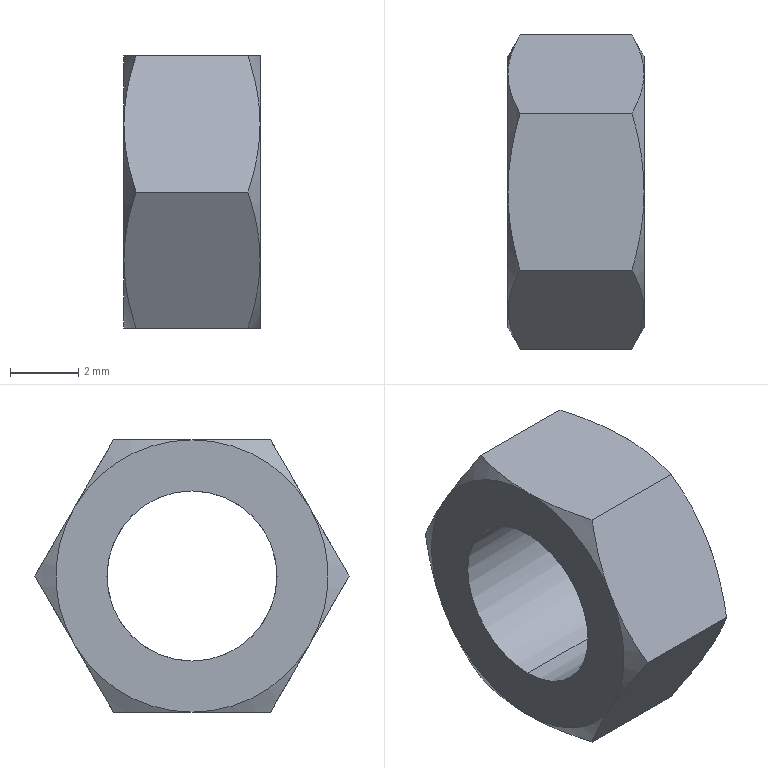Component | SolidWorks | 17268PB16x60SU(58)+(CS1-M-2)-1_17268164nut1-1 | 1 solid | 22 faces | box 4 x 9.24 x 8 mm | volume 142 mm3 | cone 12 | plane 8 | cylinder 2 | commonest cylinder face diameters 5 x2
build123d program:
from build123d import *

# Parameters (mm, degrees)
CUT_EXTRUDE1_DEPTH              = 2
CUT_EXTRUDE1_DEPTH_BACK         = 2
SKETCH3_W                       = 16
SKETCH3_H                       = 16
THREAD_FIT_RELIEF_M5_DEPTH      = 8.303
THREAD_FIT_RELIEF_M5_DEPTH_BACK = 8.303
SKETCH1_R                       = 2.5


with BuildPart() as part:
    # Sketch1_2 → Revolve1 (revolve)
    with BuildSketch(Plane.XY, mode=Mode.PRIVATE) as revolve1_sk:
        Polygon((-2, 0), (-2, 4), (-1.538, 4.8), (1.538, 4.8), (2, 4), (2, 0), align=None)
    revolve(revolve1_sk.sketch.rotate(Axis((2, 0, 0), (-1, 0, 0)), 270), axis=Axis((2, 0, 0), (-1, 0, 0)))

    # Sketch2 → Cut-Revolve1 (revolve, cut)
    with BuildSketch(Plane.XY, mode=Mode.PRIVATE) as cut_revolve1_sk:
        Polygon((-2, 0), (-2, 2.5), (-1.567, 2.067), (1.567, 2.067), (2, 2.5), (2, 0), align=None)
    revolve(cut_revolve1_sk.sketch.rotate(Axis((2, 0, 0), (-1, 0, 0)), 270), axis=Axis((2, 0, 0), (-1, 0, 0)), mode=Mode.SUBTRACT)

    # Sketch3 → Cut-Extrude1 (cut, two sides: drawn at the far end of the back side and taken through both)
    with BuildSketch(Plane(origin=(0, 0, 0), x_dir=(0, 0, -1), z_dir=(1, 0, 0)).offset(-CUT_EXTRUDE1_DEPTH_BACK)):
        Rectangle(SKETCH3_W, SKETCH3_H)
        Polygon((-4, -2.309), (0, -4.619), (4, -2.309), (4, 2.309), (0, 4.619), (-4, 2.309), align=None, mode=Mode.SUBTRACT)
    extrude(amount=CUT_EXTRUDE1_DEPTH + CUT_EXTRUDE1_DEPTH_BACK, mode=Mode.SUBTRACT)

    # Sketch1 → Thread fit relief M5 (cut, two sides: drawn at the far end of the back side and taken through both)
    with BuildSketch(Plane.ZY.offset(2).offset(-THREAD_FIT_RELIEF_M5_DEPTH_BACK)):
        Circle(SKETCH1_R)
    extrude(amount=THREAD_FIT_RELIEF_M5_DEPTH + THREAD_FIT_RELIEF_M5_DEPTH_BACK, mode=Mode.SUBTRACT)


solid = part.part

# Placed as in the assembly
solid = solid.moved(Location((-2.6, -27.579, 21.5), (0, 0, 0)))
STEP:
#1=CARTESIAN_POINT('',(-0.1811,-1.086,0.9449));
#2=VERTEX_POINT('',#1);
#3=CARTESIAN_POINT('',(-0.1811,-1.086,0.748));
#4=VERTEX_POINT('',#3);
#5=CARTESIAN_POINT('',(-0.1811,-1.086,0.8465));
#6=DIRECTION('',(1.,-0.,-0.));
#7=DIRECTION('',(0.,0.,-1.));
#8=AXIS2_PLACEMENT_3D('',#5,#6,#7);
#9=CIRCLE('',#8,0.09843);
#10=EDGE_CURVE('',#2,#4,#9,.T.);
#11=ORIENTED_EDGE('',*,*,#10,.F.);
#12=CARTESIAN_POINT('',(-0.02362,-1.086,0.9449));
#13=VERTEX_POINT('',#12);
#14=CARTESIAN_POINT('',(-0.1811,-1.086,0.9449));
#15=DIRECTION('',(1.,-0.,-0.));
#16=VECTOR('',#15,39.37);
#17=LINE('',#14,#16);
#18=EDGE_CURVE('',#2,#13,#17,.T.);
#19=ORIENTED_EDGE('',*,*,#18,.T.);
#20=CARTESIAN_POINT('',(-0.02362,-1.086,0.748));
#21=VERTEX_POINT('',#20);
#22=CARTESIAN_POINT('',(-0.02362,-1.086,0.9449));
#23=CARTESIAN_POINT('',(-0.02362,-1.099,0.9449));
#24=CARTESIAN_POINT('',(-0.02362,-1.112,0.9423));
#25=CARTESIAN_POINT('',(-0.02362,-1.135,0.9325));
#26=CARTESIAN_POINT('',(-0.02362,-1.146,0.9252));
#27=CARTESIAN_POINT('',(-0.02362,-1.165,0.9069));
#28=CARTESIAN_POINT('',(-0.02362,-1.172,0.896));
#29=CARTESIAN_POINT('',(-0.02362,-1.182,0.8722));
#30=CARTESIAN_POINT('',(-0.02362,-1.184,0.8593));
#31=CARTESIAN_POINT('',(-0.02362,-1.184,0.8336));
#32=CARTESIAN_POINT('',(-0.02362,-1.182,0.8207));
#33=CARTESIAN_POINT('',(-0.02362,-1.172,0.7969));
#34=CARTESIAN_POINT('',(-0.02362,-1.165,0.786));
#35=CARTESIAN_POINT('',(-0.02362,-1.146,0.7677));
#36=CARTESIAN_POINT('',(-0.02362,-1.135,0.7605));
#37=CARTESIAN_POINT('',(-0.02362,-1.112,0.7506));
#38=CARTESIAN_POINT('',(-0.02362,-1.099,0.748));
#39=CARTESIAN_POINT('',(-0.02362,-1.086,0.748));
#40=B_SPLINE_CURVE_WITH_KNOTS('',3,(#22,#23,#24,#25,#26,#27,#28,#29,#30,#31,#32,#33,#34,#35,#36,#37,#38,#39),.UNSPECIFIED.,.F.,.F.,(4,2,2,2,2,2,2,2,4),(0.5,0.5625,0.625,0.6875,0.75,0.8125,0.875,0.9375,1.),.UNSPECIFIED.);
#41=EDGE_CURVE('',#13,#21,#40,.T.);
#42=ORIENTED_EDGE('',*,*,#41,.T.);
#43=CARTESIAN_POINT('',(-0.1811,-1.086,0.748));
#44=DIRECTION('',(1.,-0.,-0.));
#45=VECTOR('',#44,39.37);
#46=LINE('',#43,#45);
#47=EDGE_CURVE('',#4,#21,#46,.T.);
#48=ORIENTED_EDGE('',*,*,#47,.F.);
#49=EDGE_LOOP('',(#11,#19,#42,#48));
#50=FACE_OUTER_BOUND('',#49,.T.);
#51=CARTESIAN_POINT('',(-0.1811,-1.086,0.8465));
#52=DIRECTION('',(1.,-0.,-0.));
#53=DIRECTION('',(0.,0.,-1.));
#54=AXIS2_PLACEMENT_3D('',#51,#52,#53);
#55=CYLINDRICAL_SURFACE('',#54,0.09843);
#56=ADVANCED_FACE('',(#50),#55,.F.);
#57=CARTESIAN_POINT('',(-0.03769,-0.9949,1.004));
#58=VERTEX_POINT('',#57);
#59=CARTESIAN_POINT('',(-0.02362,-0.9494,0.9252));
#60=VERTEX_POINT('',#59);
#61=CARTESIAN_POINT('',(-0.03769,-0.9949,1.004));
#62=CARTESIAN_POINT('',(-0.0291,-0.98,0.9782));
#63=CARTESIAN_POINT('',(-0.02362,-0.9649,0.952));
#64=CARTESIAN_POINT('',(-0.02362,-0.9494,0.9252));
#65=B_SPLINE_CURVE_WITH_KNOTS('',3,(#61,#62,#63,#64),.UNSPECIFIED.,.F.,.F.,(4,4),(0.00000024,0.002337),.UNSPECIFIED.);
#66=EDGE_CURVE('',#58,#60,#65,.T.);
#67=ORIENTED_EDGE('',*,*,#66,.F.);
#68=CARTESIAN_POINT('',(-0.02362,-1.086,1.004));
#69=VERTEX_POINT('',#68);
#70=CARTESIAN_POINT('',(-0.02362,-1.086,1.004));
#71=CARTESIAN_POINT('',(-0.02362,-1.07,1.004));
#72=CARTESIAN_POINT('',(-0.02498,-1.055,1.004));
#73=CARTESIAN_POINT('',(-0.02991,-1.024,1.004));
#74=CARTESIAN_POINT('',(-0.03344,-1.01,1.004));
#75=CARTESIAN_POINT('',(-0.03769,-0.9949,1.004));
#76=B_SPLINE_CURVE_WITH_KNOTS('',3,(#70,#71,#72,#73,#74,#75),.UNSPECIFIED.,.F.,.F.,(4,2,4),(0.006473,0.007642,0.008811),.UNSPECIFIED.);
#77=EDGE_CURVE('',#69,#58,#76,.T.);
#78=ORIENTED_EDGE('',*,*,#77,.F.);
#79=CARTESIAN_POINT('',(-0.02362,-1.086,0.8465));
#80=DIRECTION('',(1.,-0.,-0.));
#81=DIRECTION('',(-0.,0.,-1.));
#82=AXIS2_PLACEMENT_3D('',#79,#80,#81);
#83=CIRCLE('',#82,0.1575);
#84=EDGE_CURVE('',#60,#69,#83,.T.);
#85=ORIENTED_EDGE('',*,*,#84,.F.);
#86=EDGE_LOOP('',(#67,#78,#85));
#87=FACE_OUTER_BOUND('',#86,.T.);
#88=CARTESIAN_POINT('',(-0.04181,-1.086,0.8465));
#89=DIRECTION('',(-1.,0.,0.));
#90=DIRECTION('',(0.,0.,1.));
#91=AXIS2_PLACEMENT_3D('',#88,#89,#90);
#92=CONICAL_SURFACE('',#91,0.189,1.047);
#93=ADVANCED_FACE('',(#87),#92,.T.);
#94=CARTESIAN_POINT('',(-0.03769,-0.904,0.8465));
#95=VERTEX_POINT('',#94);
#96=CARTESIAN_POINT('',(-0.02362,-0.9494,0.9252));
#97=CARTESIAN_POINT('',(-0.02362,-0.9417,0.9118));
#98=CARTESIAN_POINT('',(-0.02497,-0.934,0.8985));
#99=CARTESIAN_POINT('',(-0.02987,-0.9189,0.8723));
#100=CARTESIAN_POINT('',(-0.0334,-0.9114,0.8593));
#101=CARTESIAN_POINT('',(-0.03769,-0.904,0.8465));
#102=B_SPLINE_CURVE_WITH_KNOTS('',3,(#96,#97,#98,#99,#100,#101),.UNSPECIFIED.,.F.,.F.,(4,2,4),(0.002337,0.003501,0.004665),.UNSPECIFIED.);
#103=EDGE_CURVE('',#60,#95,#102,.T.);
#104=ORIENTED_EDGE('',*,*,#103,.F.);
#105=CARTESIAN_POINT('',(-0.02362,-0.9494,0.7677));
#106=VERTEX_POINT('',#105);
#107=CARTESIAN_POINT('',(-0.02362,-1.086,0.8465));
#108=DIRECTION('',(1.,-0.,-0.));
#109=DIRECTION('',(-0.,0.,-1.));
#110=AXIS2_PLACEMENT_3D('',#107,#108,#109);
#111=CIRCLE('',#110,0.1575);
#112=EDGE_CURVE('',#106,#60,#111,.T.);
#113=ORIENTED_EDGE('',*,*,#112,.F.);
#114=CARTESIAN_POINT('',(-0.03769,-0.904,0.8465));
#115=CARTESIAN_POINT('',(-0.0291,-0.9188,0.8207));
#116=CARTESIAN_POINT('',(-0.02362,-0.9339,0.7945));
#117=CARTESIAN_POINT('',(-0.02362,-0.9494,0.7677));
#118=B_SPLINE_CURVE_WITH_KNOTS('',3,(#114,#115,#116,#117),.UNSPECIFIED.,.F.,.F.,(4,4),(0.00000024,0.002337),.UNSPECIFIED.);
#119=EDGE_CURVE('',#95,#106,#118,.T.);
#120=ORIENTED_EDGE('',*,*,#119,.F.);
#121=EDGE_LOOP('',(#104,#113,#120));
#122=FACE_OUTER_BOUND('',#121,.T.);
#123=CARTESIAN_POINT('',(-0.04181,-1.086,0.8465));
#124=DIRECTION('',(-1.,0.,0.));
#125=DIRECTION('',(0.,0.,1.));
#126=AXIS2_PLACEMENT_3D('',#123,#124,#125);
#127=CONICAL_SURFACE('',#126,0.189,1.047);
#128=ADVANCED_FACE('',(#122),#127,.T.);
#129=CARTESIAN_POINT('',(-0.03769,-0.9949,0.689));
#130=VERTEX_POINT('',#129);
#131=CARTESIAN_POINT('',(-0.02362,-0.9494,0.7677));
#132=CARTESIAN_POINT('',(-0.02362,-0.9571,0.7544));
#133=CARTESIAN_POINT('',(-0.02497,-0.9648,0.741));
#134=CARTESIAN_POINT('',(-0.02987,-0.98,0.7148));
#135=CARTESIAN_POINT('',(-0.0334,-0.9875,0.7018));
#136=CARTESIAN_POINT('',(-0.03769,-0.9949,0.689));
#137=B_SPLINE_CURVE_WITH_KNOTS('',3,(#131,#132,#133,#134,#135,#136),.UNSPECIFIED.,.F.,.F.,(4,2,4),(0.002337,0.003501,0.004665),.UNSPECIFIED.);
#138=EDGE_CURVE('',#106,#130,#137,.T.);
#139=ORIENTED_EDGE('',*,*,#138,.F.);
#140=CARTESIAN_POINT('',(-0.02362,-1.086,0.689));
#141=VERTEX_POINT('',#140);
#142=CARTESIAN_POINT('',(-0.02362,-1.086,0.8465));
#143=DIRECTION('',(1.,-0.,-0.));
#144=DIRECTION('',(-0.,0.,-1.));
#145=AXIS2_PLACEMENT_3D('',#142,#143,#144);
#146=CIRCLE('',#145,0.1575);
#147=EDGE_CURVE('',#141,#106,#146,.T.);
#148=ORIENTED_EDGE('',*,*,#147,.F.);
#149=CARTESIAN_POINT('',(-0.03769,-0.9949,0.689));
#150=CARTESIAN_POINT('',(-0.03344,-1.01,0.689));
#151=CARTESIAN_POINT('',(-0.02991,-1.024,0.689));
#152=CARTESIAN_POINT('',(-0.02498,-1.055,0.689));
#153=CARTESIAN_POINT('',(-0.02362,-1.07,0.689));
#154=CARTESIAN_POINT('',(-0.02362,-1.086,0.689));
#155=B_SPLINE_CURVE_WITH_KNOTS('',3,(#149,#150,#151,#152,#153,#154),.UNSPECIFIED.,.F.,.F.,(4,2,4),(0.01014,0.01131,0.01248),.UNSPECIFIED.);
#156=EDGE_CURVE('',#130,#141,#155,.T.);
#157=ORIENTED_EDGE('',*,*,#156,.F.);
#158=EDGE_LOOP('',(#139,#148,#157));
#159=FACE_OUTER_BOUND('',#158,.T.);
#160=CARTESIAN_POINT('',(-0.04181,-1.086,0.8465));
#161=DIRECTION('',(-1.,0.,0.));
#162=DIRECTION('',(0.,0.,1.));
#163=AXIS2_PLACEMENT_3D('',#160,#161,#162);
#164=CONICAL_SURFACE('',#163,0.189,1.047);
#165=ADVANCED_FACE('',(#159),#164,.T.);
#166=CARTESIAN_POINT('',(-0.03769,-1.177,1.004));
#167=VERTEX_POINT('',#166);
#168=CARTESIAN_POINT('',(-0.03769,-1.177,1.004));
#169=CARTESIAN_POINT('',(-0.03342,-1.162,1.004));
#170=CARTESIAN_POINT('',(-0.02984,-1.147,1.004));
#171=CARTESIAN_POINT('',(-0.02494,-1.116,1.004));
#172=CARTESIAN_POINT('',(-0.02362,-1.101,1.004));
#173=CARTESIAN_POINT('',(-0.02362,-1.086,1.004));
#174=B_SPLINE_CURVE_WITH_KNOTS('',3,(#168,#169,#170,#171,#172,#173),.UNSPECIFIED.,.F.,.F.,(4,2,4),(0.004136,0.005305,0.006473),.UNSPECIFIED.);
#175=EDGE_CURVE('',#167,#69,#174,.T.);
#176=ORIENTED_EDGE('',*,*,#175,.F.);
#177=CARTESIAN_POINT('',(-0.02362,-1.222,0.9252));
#178=VERTEX_POINT('',#177);
#179=CARTESIAN_POINT('',(-0.02362,-1.222,0.9252));
#180=CARTESIAN_POINT('',(-0.02362,-1.214,0.9386));
#181=CARTESIAN_POINT('',(-0.02497,-1.207,0.9519));
#182=CARTESIAN_POINT('',(-0.02987,-1.192,0.9781));
#183=CARTESIAN_POINT('',(-0.0334,-1.184,0.9911));
#184=CARTESIAN_POINT('',(-0.03769,-1.177,1.004));
#185=B_SPLINE_CURVE_WITH_KNOTS('',3,(#179,#180,#181,#182,#183,#184),.UNSPECIFIED.,.F.,.F.,(4,2,4),(0.002337,0.003501,0.004665),.UNSPECIFIED.);
#186=EDGE_CURVE('',#178,#167,#185,.T.);
#187=ORIENTED_EDGE('',*,*,#186,.F.);
#188=CARTESIAN_POINT('',(-0.02362,-1.086,0.8465));
#189=DIRECTION('',(1.,-0.,-0.));
#190=DIRECTION('',(-0.,0.,-1.));
#191=AXIS2_PLACEMENT_3D('',#188,#189,#190);
#192=CIRCLE('',#191,0.1575);
#193=EDGE_CURVE('',#69,#178,#192,.T.);
#194=ORIENTED_EDGE('',*,*,#193,.F.);
#195=EDGE_LOOP('',(#176,#187,#194));
#196=FACE_OUTER_BOUND('',#195,.T.);
#197=CARTESIAN_POINT('',(-0.04181,-1.086,0.8465));
#198=DIRECTION('',(-1.,0.,0.));
#199=DIRECTION('',(0.,0.,1.));
#200=AXIS2_PLACEMENT_3D('',#197,#198,#199);
#201=CONICAL_SURFACE('',#200,0.189,1.047);
#202=ADVANCED_FACE('',(#196),#201,.T.);
#203=CARTESIAN_POINT('',(-0.03769,-1.177,0.689));
#204=VERTEX_POINT('',#203);
#205=CARTESIAN_POINT('',(-0.02362,-1.086,0.689));
#206=CARTESIAN_POINT('',(-0.02362,-1.101,0.689));
#207=CARTESIAN_POINT('',(-0.02494,-1.116,0.689));
#208=CARTESIAN_POINT('',(-0.02984,-1.147,0.689));
#209=CARTESIAN_POINT('',(-0.03342,-1.162,0.689));
#210=CARTESIAN_POINT('',(-0.03769,-1.177,0.689));
#211=B_SPLINE_CURVE_WITH_KNOTS('',3,(#205,#206,#207,#208,#209,#210),.UNSPECIFIED.,.F.,.F.,(4,2,4),(0.01248,0.01365,0.01482),.UNSPECIFIED.);
#212=EDGE_CURVE('',#141,#204,#211,.T.);
#213=ORIENTED_EDGE('',*,*,#212,.F.);
#214=CARTESIAN_POINT('',(-0.02362,-1.222,0.7677));
#215=VERTEX_POINT('',#214);
#216=CARTESIAN_POINT('',(-0.02362,-1.086,0.8465));
#217=DIRECTION('',(1.,-0.,-0.));
#218=DIRECTION('',(-0.,0.,-1.));
#219=AXIS2_PLACEMENT_3D('',#216,#217,#218);
#220=CIRCLE('',#219,0.1575);
#221=EDGE_CURVE('',#215,#141,#220,.T.);
#222=ORIENTED_EDGE('',*,*,#221,.F.);
#223=CARTESIAN_POINT('',(-0.03769,-1.177,0.689));
#224=CARTESIAN_POINT('',(-0.0291,-1.192,0.7147));
#225=CARTESIAN_POINT('',(-0.02362,-1.207,0.7409));
#226=CARTESIAN_POINT('',(-0.02362,-1.222,0.7677));
#227=B_SPLINE_CURVE_WITH_KNOTS('',3,(#223,#224,#225,#226),.UNSPECIFIED.,.F.,.F.,(4,4),(0.00000024,0.002337),.UNSPECIFIED.);
#228=EDGE_CURVE('',#204,#215,#227,.T.);
#229=ORIENTED_EDGE('',*,*,#228,.F.);
#230=EDGE_LOOP('',(#213,#222,#229));
#231=FACE_OUTER_BOUND('',#230,.T.);
#232=CARTESIAN_POINT('',(-0.04181,-1.086,0.8465));
#233=DIRECTION('',(-1.,0.,0.));
#234=DIRECTION('',(0.,0.,1.));
#235=AXIS2_PLACEMENT_3D('',#232,#233,#234);
#236=CONICAL_SURFACE('',#235,0.189,1.047);
#237=ADVANCED_FACE('',(#231),#236,.T.);
#238=CARTESIAN_POINT('',(-0.03769,-1.268,0.8465));
#239=VERTEX_POINT('',#238);
#240=CARTESIAN_POINT('',(-0.03769,-1.268,0.8465));
#241=CARTESIAN_POINT('',(-0.0291,-1.253,0.8722));
#242=CARTESIAN_POINT('',(-0.02362,-1.238,0.8984));
#243=CARTESIAN_POINT('',(-0.02362,-1.222,0.9252));
#244=B_SPLINE_CURVE_WITH_KNOTS('',3,(#240,#241,#242,#243),.UNSPECIFIED.,.F.,.F.,(4,4),(0.00000024,0.002337),.UNSPECIFIED.);
#245=EDGE_CURVE('',#239,#178,#244,.T.);
#246=ORIENTED_EDGE('',*,*,#245,.F.);
#247=CARTESIAN_POINT('',(-0.02362,-1.222,0.7677));
#248=CARTESIAN_POINT('',(-0.02362,-1.23,0.7811));
#249=CARTESIAN_POINT('',(-0.02497,-1.238,0.7944));
#250=CARTESIAN_POINT('',(-0.02987,-1.253,0.8207));
#251=CARTESIAN_POINT('',(-0.0334,-1.26,0.8336));
#252=CARTESIAN_POINT('',(-0.03769,-1.268,0.8465));
#253=B_SPLINE_CURVE_WITH_KNOTS('',3,(#247,#248,#249,#250,#251,#252),.UNSPECIFIED.,.F.,.F.,(4,2,4),(0.002337,0.003501,0.004665),.UNSPECIFIED.);
#254=EDGE_CURVE('',#215,#239,#253,.T.);
#255=ORIENTED_EDGE('',*,*,#254,.F.);
#256=CARTESIAN_POINT('',(-0.02362,-1.086,0.8465));
#257=DIRECTION('',(1.,-0.,-0.));
#258=DIRECTION('',(-0.,0.,-1.));
#259=AXIS2_PLACEMENT_3D('',#256,#257,#258);
#260=CIRCLE('',#259,0.1575);
#261=EDGE_CURVE('',#178,#215,#260,.T.);
#262=ORIENTED_EDGE('',*,*,#261,.F.);
#263=EDGE_LOOP('',(#246,#255,#262));
#264=FACE_OUTER_BOUND('',#263,.T.);
#265=CARTESIAN_POINT('',(-0.04181,-1.086,0.8465));
#266=DIRECTION('',(-1.,0.,0.));
#267=DIRECTION('',(0.,0.,1.));
#268=AXIS2_PLACEMENT_3D('',#265,#266,#267);
#269=CONICAL_SURFACE('',#268,0.189,1.047);
#270=ADVANCED_FACE('',(#264),#269,.T.);
#271=CARTESIAN_POINT('',(-0.167,-1.177,0.689));
#272=VERTEX_POINT('',#271);
#273=CARTESIAN_POINT('',(-0.1811,-1.086,0.689));
#274=VERTEX_POINT('',#273);
#275=CARTESIAN_POINT('',(-0.167,-1.177,0.689));
#276=CARTESIAN_POINT('',(-0.1713,-1.162,0.689));
#277=CARTESIAN_POINT('',(-0.1749,-1.147,0.689));
#278=CARTESIAN_POINT('',(-0.1798,-1.116,0.689));
#279=CARTESIAN_POINT('',(-0.1811,-1.101,0.689));
#280=CARTESIAN_POINT('',(-0.1811,-1.086,0.689));
#281=B_SPLINE_CURVE_WITH_KNOTS('',3,(#275,#276,#277,#278,#279,#280),.UNSPECIFIED.,.F.,.F.,(4,2,4),(0.004136,0.005305,0.006473),.UNSPECIFIED.);
#282=EDGE_CURVE('',#272,#274,#281,.T.);
#283=ORIENTED_EDGE('',*,*,#282,.F.);
#284=CARTESIAN_POINT('',(-0.1811,-1.222,0.7677));
#285=VERTEX_POINT('',#284);
#286=CARTESIAN_POINT('',(-0.1811,-1.222,0.7677));
#287=CARTESIAN_POINT('',(-0.1811,-1.214,0.7544));
#288=CARTESIAN_POINT('',(-0.1798,-1.207,0.741));
#289=CARTESIAN_POINT('',(-0.1749,-1.192,0.7148));
#290=CARTESIAN_POINT('',(-0.1713,-1.184,0.7018));
#291=CARTESIAN_POINT('',(-0.167,-1.177,0.689));
#292=B_SPLINE_CURVE_WITH_KNOTS('',3,(#286,#287,#288,#289,#290,#291),.UNSPECIFIED.,.F.,.F.,(4,2,4),(0.002337,0.003501,0.004665),.UNSPECIFIED.);
#293=EDGE_CURVE('',#285,#272,#292,.T.);
#294=ORIENTED_EDGE('',*,*,#293,.F.);
#295=CARTESIAN_POINT('',(-0.1811,-1.086,0.8465));
#296=DIRECTION('',(1.,-0.,-0.));
#297=DIRECTION('',(0.,0.,-1.));
#298=AXIS2_PLACEMENT_3D('',#295,#296,#297);
#299=CIRCLE('',#298,0.1575);
#300=EDGE_CURVE('',#285,#274,#299,.T.);
#301=ORIENTED_EDGE('',*,*,#300,.T.);
#302=EDGE_LOOP('',(#283,#294,#301));
#303=FACE_OUTER_BOUND('',#302,.T.);
#304=CARTESIAN_POINT('',(-0.1811,-1.086,0.8465));
#305=DIRECTION('',(1.,-0.,-0.));
#306=DIRECTION('',(0.,0.,-1.));
#307=AXIS2_PLACEMENT_3D('',#304,#305,#306);
#308=CONICAL_SURFACE('',#307,0.1575,1.047);
#309=ADVANCED_FACE('',(#303),#308,.T.);
#310=CARTESIAN_POINT('',(-0.167,-0.9949,0.689));
#311=VERTEX_POINT('',#310);
#312=CARTESIAN_POINT('',(-0.1811,-1.086,0.689));
#313=CARTESIAN_POINT('',(-0.1811,-1.07,0.689));
#314=CARTESIAN_POINT('',(-0.1797,-1.055,0.689));
#315=CARTESIAN_POINT('',(-0.1748,-1.024,0.689));
#316=CARTESIAN_POINT('',(-0.1713,-1.01,0.689));
#317=CARTESIAN_POINT('',(-0.167,-0.9949,0.689));
#318=B_SPLINE_CURVE_WITH_KNOTS('',3,(#312,#313,#314,#315,#316,#317),.UNSPECIFIED.,.F.,.F.,(4,2,4),(0.006473,0.007642,0.008811),.UNSPECIFIED.);
#319=EDGE_CURVE('',#274,#311,#318,.T.);
#320=ORIENTED_EDGE('',*,*,#319,.F.);
#321=CARTESIAN_POINT('',(-0.1811,-0.9494,0.7677));
#322=VERTEX_POINT('',#321);
#323=CARTESIAN_POINT('',(-0.1811,-1.086,0.8465));
#324=DIRECTION('',(1.,-0.,-0.));
#325=DIRECTION('',(0.,0.,-1.));
#326=AXIS2_PLACEMENT_3D('',#323,#324,#325);
#327=CIRCLE('',#326,0.1575);
#328=EDGE_CURVE('',#274,#322,#327,.T.);
#329=ORIENTED_EDGE('',*,*,#328,.T.);
#330=CARTESIAN_POINT('',(-0.167,-0.9949,0.689));
#331=CARTESIAN_POINT('',(-0.1756,-0.98,0.7147));
#332=CARTESIAN_POINT('',(-0.1811,-0.9649,0.7409));
#333=CARTESIAN_POINT('',(-0.1811,-0.9494,0.7677));
#334=B_SPLINE_CURVE_WITH_KNOTS('',3,(#330,#331,#332,#333),.UNSPECIFIED.,.F.,.F.,(4,4),(0.00000024,0.002337),.UNSPECIFIED.);
#335=EDGE_CURVE('',#311,#322,#334,.T.);
#336=ORIENTED_EDGE('',*,*,#335,.F.);
#337=EDGE_LOOP('',(#320,#329,#336));
#338=FACE_OUTER_BOUND('',#337,.T.);
#339=CARTESIAN_POINT('',(-0.1811,-1.086,0.8465));
#340=DIRECTION('',(1.,-0.,-0.));
#341=DIRECTION('',(0.,0.,-1.));
#342=AXIS2_PLACEMENT_3D('',#339,#340,#341);
#343=CONICAL_SURFACE('',#342,0.1575,1.047);
#344=ADVANCED_FACE('',(#338),#343,.T.);
#345=CARTESIAN_POINT('',(-0.167,-0.904,0.8465));
#346=VERTEX_POINT('',#345);
#347=CARTESIAN_POINT('',(-0.1811,-0.9494,0.7677));
#348=CARTESIAN_POINT('',(-0.1811,-0.9417,0.7811));
#349=CARTESIAN_POINT('',(-0.1798,-0.934,0.7944));
#350=CARTESIAN_POINT('',(-0.1749,-0.9189,0.8207));
#351=CARTESIAN_POINT('',(-0.1713,-0.9114,0.8336));
#352=CARTESIAN_POINT('',(-0.167,-0.904,0.8465));
#353=B_SPLINE_CURVE_WITH_KNOTS('',3,(#347,#348,#349,#350,#351,#352),.UNSPECIFIED.,.F.,.F.,(4,2,4),(0.002337,0.003501,0.004665),.UNSPECIFIED.);
#354=EDGE_CURVE('',#322,#346,#353,.T.);
#355=ORIENTED_EDGE('',*,*,#354,.F.);
#356=CARTESIAN_POINT('',(-0.1811,-0.9494,0.9252));
#357=VERTEX_POINT('',#356);
#358=CARTESIAN_POINT('',(-0.1811,-1.086,0.8465));
#359=DIRECTION('',(1.,-0.,-0.));
#360=DIRECTION('',(0.,0.,-1.));
#361=AXIS2_PLACEMENT_3D('',#358,#359,#360);
#362=CIRCLE('',#361,0.1575);
#363=EDGE_CURVE('',#322,#357,#362,.T.);
#364=ORIENTED_EDGE('',*,*,#363,.T.);
#365=CARTESIAN_POINT('',(-0.167,-0.904,0.8465));
#366=CARTESIAN_POINT('',(-0.1756,-0.9188,0.8722));
#367=CARTESIAN_POINT('',(-0.1811,-0.9339,0.8984));
#368=CARTESIAN_POINT('',(-0.1811,-0.9494,0.9252));
#369=B_SPLINE_CURVE_WITH_KNOTS('',3,(#365,#366,#367,#368),.UNSPECIFIED.,.F.,.F.,(4,4),(0.00000024,0.002337),.UNSPECIFIED.);
#370=EDGE_CURVE('',#346,#357,#369,.T.);
#371=ORIENTED_EDGE('',*,*,#370,.F.);
#372=EDGE_LOOP('',(#355,#364,#371));
#373=FACE_OUTER_BOUND('',#372,.T.);
#374=CARTESIAN_POINT('',(-0.1811,-1.086,0.8465));
#375=DIRECTION('',(1.,-0.,-0.));
#376=DIRECTION('',(0.,0.,-1.));
#377=AXIS2_PLACEMENT_3D('',#374,#375,#376);
#378=CONICAL_SURFACE('',#377,0.1575,1.047);
#379=ADVANCED_FACE('',(#373),#378,.T.);
#380=CARTESIAN_POINT('',(-0.167,-0.9949,1.004));
#381=VERTEX_POINT('',#380);
#382=CARTESIAN_POINT('',(-0.1811,-0.9494,0.9252));
#383=CARTESIAN_POINT('',(-0.1811,-0.9571,0.9386));
#384=CARTESIAN_POINT('',(-0.1798,-0.9648,0.9519));
#385=CARTESIAN_POINT('',(-0.1749,-0.98,0.9781));
#386=CARTESIAN_POINT('',(-0.1713,-0.9875,0.9911));
#387=CARTESIAN_POINT('',(-0.167,-0.9949,1.004));
#388=B_SPLINE_CURVE_WITH_KNOTS('',3,(#382,#383,#384,#385,#386,#387),.UNSPECIFIED.,.F.,.F.,(4,2,4),(0.002337,0.003501,0.004665),.UNSPECIFIED.);
#389=EDGE_CURVE('',#357,#381,#388,.T.);
#390=ORIENTED_EDGE('',*,*,#389,.F.);
#391=CARTESIAN_POINT('',(-0.1811,-1.086,1.004));
#392=VERTEX_POINT('',#391);
#393=CARTESIAN_POINT('',(-0.1811,-1.086,0.8465));
#394=DIRECTION('',(1.,-0.,-0.));
#395=DIRECTION('',(0.,0.,-1.));
#396=AXIS2_PLACEMENT_3D('',#393,#394,#395);
#397=CIRCLE('',#396,0.1575);
#398=EDGE_CURVE('',#357,#392,#397,.T.);
#399=ORIENTED_EDGE('',*,*,#398,.T.);
#400=CARTESIAN_POINT('',(-0.167,-0.9949,1.004));
#401=CARTESIAN_POINT('',(-0.1713,-1.01,1.004));
#402=CARTESIAN_POINT('',(-0.1748,-1.024,1.004));
#403=CARTESIAN_POINT('',(-0.1797,-1.055,1.004));
#404=CARTESIAN_POINT('',(-0.1811,-1.07,1.004));
#405=CARTESIAN_POINT('',(-0.1811,-1.086,1.004));
#406=B_SPLINE_CURVE_WITH_KNOTS('',3,(#400,#401,#402,#403,#404,#405),.UNSPECIFIED.,.F.,.F.,(4,2,4),(0.01014,0.01131,0.01248),.UNSPECIFIED.);
#407=EDGE_CURVE('',#381,#392,#406,.T.);
#408=ORIENTED_EDGE('',*,*,#407,.F.);
#409=EDGE_LOOP('',(#390,#399,#408));
#410=FACE_OUTER_BOUND('',#409,.T.);
#411=CARTESIAN_POINT('',(-0.1811,-1.086,0.8465));
#412=DIRECTION('',(1.,-0.,-0.));
#413=DIRECTION('',(0.,0.,-1.));
#414=AXIS2_PLACEMENT_3D('',#411,#412,#413);
#415=CONICAL_SURFACE('',#414,0.1575,1.047);
#416=ADVANCED_FACE('',(#410),#415,.T.);
#417=CARTESIAN_POINT('',(-0.167,-1.177,1.004));
#418=VERTEX_POINT('',#417);
#419=CARTESIAN_POINT('',(-0.1811,-1.086,1.004));
#420=CARTESIAN_POINT('',(-0.1811,-1.101,1.004));
#421=CARTESIAN_POINT('',(-0.1798,-1.116,1.004));
#422=CARTESIAN_POINT('',(-0.1749,-1.147,1.004));
#423=CARTESIAN_POINT('',(-0.1713,-1.162,1.004));
#424=CARTESIAN_POINT('',(-0.167,-1.177,1.004));
#425=B_SPLINE_CURVE_WITH_KNOTS('',3,(#419,#420,#421,#422,#423,#424),.UNSPECIFIED.,.F.,.F.,(4,2,4),(0.01248,0.01365,0.01482),.UNSPECIFIED.);
#426=EDGE_CURVE('',#392,#418,#425,.T.);
#427=ORIENTED_EDGE('',*,*,#426,.F.);
#428=CARTESIAN_POINT('',(-0.1811,-1.222,0.9252));
#429=VERTEX_POINT('',#428);
#430=CARTESIAN_POINT('',(-0.1811,-1.086,0.8465));
#431=DIRECTION('',(1.,-0.,-0.));
#432=DIRECTION('',(0.,0.,-1.));
#433=AXIS2_PLACEMENT_3D('',#430,#431,#432);
#434=CIRCLE('',#433,0.1575);
#435=EDGE_CURVE('',#392,#429,#434,.T.);
#436=ORIENTED_EDGE('',*,*,#435,.T.);
#437=CARTESIAN_POINT('',(-0.167,-1.177,1.004));
#438=CARTESIAN_POINT('',(-0.1756,-1.192,0.9782));
#439=CARTESIAN_POINT('',(-0.1811,-1.207,0.952));
#440=CARTESIAN_POINT('',(-0.1811,-1.222,0.9252));
#441=B_SPLINE_CURVE_WITH_KNOTS('',3,(#437,#438,#439,#440),.UNSPECIFIED.,.F.,.F.,(4,4),(0.00000024,0.002337),.UNSPECIFIED.);
#442=EDGE_CURVE('',#418,#429,#441,.T.);
#443=ORIENTED_EDGE('',*,*,#442,.F.);
#444=EDGE_LOOP('',(#427,#436,#443));
#445=FACE_OUTER_BOUND('',#444,.T.);
#446=CARTESIAN_POINT('',(-0.1811,-1.086,0.8465));
#447=DIRECTION('',(1.,-0.,-0.));
#448=DIRECTION('',(0.,0.,-1.));
#449=AXIS2_PLACEMENT_3D('',#446,#447,#448);
#450=CONICAL_SURFACE('',#449,0.1575,1.047);
#451=ADVANCED_FACE('',(#445),#450,.T.);
#452=CARTESIAN_POINT('',(-0.167,-1.268,0.8465));
#453=VERTEX_POINT('',#452);
#454=CARTESIAN_POINT('',(-0.1811,-1.222,0.9252));
#455=CARTESIAN_POINT('',(-0.1811,-1.23,0.9118));
#456=CARTESIAN_POINT('',(-0.1798,-1.238,0.8985));
#457=CARTESIAN_POINT('',(-0.1749,-1.253,0.8723));
#458=CARTESIAN_POINT('',(-0.1713,-1.26,0.8593));
#459=CARTESIAN_POINT('',(-0.167,-1.268,0.8465));
#460=B_SPLINE_CURVE_WITH_KNOTS('',3,(#454,#455,#456,#457,#458,#459),.UNSPECIFIED.,.F.,.F.,(4,2,4),(0.002337,0.003501,0.004665),.UNSPECIFIED.);
#461=EDGE_CURVE('',#429,#453,#460,.T.);
#462=ORIENTED_EDGE('',*,*,#461,.F.);
#463=CARTESIAN_POINT('',(-0.1811,-1.086,0.8465));
#464=DIRECTION('',(1.,-0.,-0.));
#465=DIRECTION('',(0.,0.,-1.));
#466=AXIS2_PLACEMENT_3D('',#463,#464,#465);
#467=CIRCLE('',#466,0.1575);
#468=EDGE_CURVE('',#429,#285,#467,.T.);
#469=ORIENTED_EDGE('',*,*,#468,.T.);
#470=CARTESIAN_POINT('',(-0.167,-1.268,0.8465));
#471=CARTESIAN_POINT('',(-0.1756,-1.253,0.8207));
#472=CARTESIAN_POINT('',(-0.1811,-1.238,0.7945));
#473=CARTESIAN_POINT('',(-0.1811,-1.222,0.7677));
#474=B_SPLINE_CURVE_WITH_KNOTS('',3,(#470,#471,#472,#473),.UNSPECIFIED.,.F.,.F.,(4,4),(0.00000024,0.002337),.UNSPECIFIED.);
#475=EDGE_CURVE('',#453,#285,#474,.T.);
#476=ORIENTED_EDGE('',*,*,#475,.F.);
#477=EDGE_LOOP('',(#462,#469,#476));
#478=FACE_OUTER_BOUND('',#477,.T.);
#479=CARTESIAN_POINT('',(-0.1811,-1.086,0.8465));
#480=DIRECTION('',(1.,-0.,-0.));
#481=DIRECTION('',(0.,0.,-1.));
#482=AXIS2_PLACEMENT_3D('',#479,#480,#481);
#483=CONICAL_SURFACE('',#482,0.1575,1.047);
#484=ADVANCED_FACE('',(#478),#483,.T.);
#485=CARTESIAN_POINT('',(-0.02362,-1.086,0.748));
#486=CARTESIAN_POINT('',(-0.02362,-1.073,0.748));
#487=CARTESIAN_POINT('',(-0.02362,-1.06,0.7506));
#488=CARTESIAN_POINT('',(-0.02362,-1.036,0.7605));
#489=CARTESIAN_POINT('',(-0.02362,-1.025,0.7677));
#490=CARTESIAN_POINT('',(-0.02362,-1.007,0.786));
#491=CARTESIAN_POINT('',(-0.02362,-0.9998,0.7969));
#492=CARTESIAN_POINT('',(-0.02362,-0.9899,0.8207));
#493=CARTESIAN_POINT('',(-0.02362,-0.9874,0.8336));
#494=CARTESIAN_POINT('',(-0.02362,-0.9874,0.8593));
#495=CARTESIAN_POINT('',(-0.02362,-0.9899,0.8722));
#496=CARTESIAN_POINT('',(-0.02362,-0.9998,0.896));
#497=CARTESIAN_POINT('',(-0.02362,-1.007,0.9069));
#498=CARTESIAN_POINT('',(-0.02362,-1.025,0.9252));
#499=CARTESIAN_POINT('',(-0.02362,-1.036,0.9325));
#500=CARTESIAN_POINT('',(-0.02362,-1.06,0.9423));
#501=CARTESIAN_POINT('',(-0.02362,-1.073,0.9449));
#502=CARTESIAN_POINT('',(-0.02362,-1.086,0.9449));
#503=B_SPLINE_CURVE_WITH_KNOTS('',3,(#485,#486,#487,#488,#489,#490,#491,#492,#493,#494,#495,#496,#497,#498,#499,#500,#501,#502),.UNSPECIFIED.,.F.,.F.,(4,2,2,2,2,2,2,2,4),(0.,0.0625,0.125,0.1875,0.25,0.3125,0.375,0.4375,0.5),.UNSPECIFIED.);
#504=EDGE_CURVE('',#21,#13,#503,.T.);
#505=ORIENTED_EDGE('',*,*,#504,.F.);
#506=ORIENTED_EDGE('',*,*,#41,.F.);
#507=EDGE_LOOP('',(#505,#506));
#508=FACE_BOUND('',#507,.T.);
#509=ORIENTED_EDGE('',*,*,#147,.T.);
#510=ORIENTED_EDGE('',*,*,#112,.T.);
#511=ORIENTED_EDGE('',*,*,#84,.T.);
#512=ORIENTED_EDGE('',*,*,#193,.T.);
#513=ORIENTED_EDGE('',*,*,#261,.T.);
#514=ORIENTED_EDGE('',*,*,#221,.T.);
#515=EDGE_LOOP('',(#509,#510,#511,#512,#513,#514));
#516=FACE_OUTER_BOUND('',#515,.T.);
#517=CARTESIAN_POINT('',(-0.02362,-1.086,0.8465));
#518=DIRECTION('',(-1.,0.,0.));
#519=DIRECTION('',(0.,0.,1.));
#520=AXIS2_PLACEMENT_3D('',#517,#518,#519);
#521=PLANE('',#520);
#522=ADVANCED_FACE('',(#508,#516),#521,.F.);
#523=CARTESIAN_POINT('',(-0.1811,-1.086,0.8465));
#524=DIRECTION('',(1.,-0.,-0.));
#525=DIRECTION('',(0.,0.,-1.));
#526=AXIS2_PLACEMENT_3D('',#523,#524,#525);
#527=CIRCLE('',#526,0.09843);
#528=EDGE_CURVE('',#4,#2,#527,.T.);
#529=ORIENTED_EDGE('',*,*,#528,.T.);
#530=ORIENTED_EDGE('',*,*,#10,.T.);
#531=EDGE_LOOP('',(#529,#530));
#532=FACE_BOUND('',#531,.T.);
#533=ORIENTED_EDGE('',*,*,#328,.F.);
#534=ORIENTED_EDGE('',*,*,#300,.F.);
#535=ORIENTED_EDGE('',*,*,#468,.F.);
#536=ORIENTED_EDGE('',*,*,#435,.F.);
#537=ORIENTED_EDGE('',*,*,#398,.F.);
#538=ORIENTED_EDGE('',*,*,#363,.F.);
#539=EDGE_LOOP('',(#533,#534,#535,#536,#537,#538));
#540=FACE_OUTER_BOUND('',#539,.T.);
#541=CARTESIAN_POINT('',(-0.1811,-0.9283,0.8465));
#542=DIRECTION('',(1.,-0.,-0.));
#543=DIRECTION('',(-0.,0.,-1.));
#544=AXIS2_PLACEMENT_3D('',#541,#542,#543);
#545=PLANE('',#544);
#546=ADVANCED_FACE('',(#532,#540),#545,.F.);
#547=ORIENTED_EDGE('',*,*,#156,.T.);
#548=ORIENTED_EDGE('',*,*,#212,.T.);
#549=CARTESIAN_POINT('',(-0.02362,-1.177,0.689));
#550=DIRECTION('',(-1.,0.,0.));
#551=VECTOR('',#550,39.37);
#552=LINE('',#549,#551);
#553=EDGE_CURVE('',#204,#272,#552,.T.);
#554=ORIENTED_EDGE('',*,*,#553,.T.);
#555=ORIENTED_EDGE('',*,*,#282,.T.);
#556=ORIENTED_EDGE('',*,*,#319,.T.);
#557=CARTESIAN_POINT('',(-0.02362,-0.9949,0.689));
#558=DIRECTION('',(-1.,0.,0.));
#559=VECTOR('',#558,39.37);
#560=LINE('',#557,#559);
#561=EDGE_CURVE('',#130,#311,#560,.T.);
#562=ORIENTED_EDGE('',*,*,#561,.F.);
#563=EDGE_LOOP('',(#547,#548,#554,#555,#556,#562));
#564=FACE_OUTER_BOUND('',#563,.T.);
#565=CARTESIAN_POINT('',(-0.02362,-0.9949,0.689));
#566=DIRECTION('',(-0.,0.,-1.));
#567=DIRECTION('',(-1.,0.,0.));
#568=AXIS2_PLACEMENT_3D('',#565,#566,#567);
#569=PLANE('',#568);
#570=ADVANCED_FACE('',(#564),#569,.T.);
#571=ORIENTED_EDGE('',*,*,#119,.T.);
#572=ORIENTED_EDGE('',*,*,#138,.T.);
#573=ORIENTED_EDGE('',*,*,#561,.T.);
#574=ORIENTED_EDGE('',*,*,#335,.T.);
#575=ORIENTED_EDGE('',*,*,#354,.T.);
#576=CARTESIAN_POINT('',(-0.02362,-0.904,0.8465));
#577=DIRECTION('',(-1.,0.,0.));
#578=VECTOR('',#577,39.37);
#579=LINE('',#576,#578);
#580=EDGE_CURVE('',#95,#346,#579,.T.);
#581=ORIENTED_EDGE('',*,*,#580,.F.);
#582=EDGE_LOOP('',(#571,#572,#573,#574,#575,#581));
#583=FACE_OUTER_BOUND('',#582,.T.);
#584=CARTESIAN_POINT('',(-0.02362,-0.904,0.8465));
#585=DIRECTION('',(-0.,0.866,-0.5));
#586=DIRECTION('',(-0.,-0.5,-0.866));
#587=AXIS2_PLACEMENT_3D('',#584,#585,#586);
#588=PLANE('',#587);
#589=ADVANCED_FACE('',(#583),#588,.T.);
#590=ORIENTED_EDGE('',*,*,#66,.T.);
#591=ORIENTED_EDGE('',*,*,#103,.T.);
#592=ORIENTED_EDGE('',*,*,#580,.T.);
#593=ORIENTED_EDGE('',*,*,#370,.T.);
#594=ORIENTED_EDGE('',*,*,#389,.T.);
#595=CARTESIAN_POINT('',(-0.02362,-0.9949,1.004));
#596=DIRECTION('',(-1.,0.,0.));
#597=VECTOR('',#596,39.37);
#598=LINE('',#595,#597);
#599=EDGE_CURVE('',#58,#381,#598,.T.);
#600=ORIENTED_EDGE('',*,*,#599,.F.);
#601=EDGE_LOOP('',(#590,#591,#592,#593,#594,#600));
#602=FACE_OUTER_BOUND('',#601,.T.);
#603=CARTESIAN_POINT('',(-0.02362,-0.9949,1.004));
#604=DIRECTION('',(0.,0.866,0.5));
#605=DIRECTION('',(-0.,0.5,-0.866));
#606=AXIS2_PLACEMENT_3D('',#603,#604,#605);
#607=PLANE('',#606);
#608=ADVANCED_FACE('',(#602),#607,.T.);
#609=ORIENTED_EDGE('',*,*,#175,.T.);
#610=ORIENTED_EDGE('',*,*,#77,.T.);
#611=ORIENTED_EDGE('',*,*,#599,.T.);
#612=ORIENTED_EDGE('',*,*,#407,.T.);
#613=ORIENTED_EDGE('',*,*,#426,.T.);
#614=CARTESIAN_POINT('',(-0.02362,-1.177,1.004));
#615=DIRECTION('',(-1.,0.,0.));
#616=VECTOR('',#615,39.37);
#617=LINE('',#614,#616);
#618=EDGE_CURVE('',#167,#418,#617,.T.);
#619=ORIENTED_EDGE('',*,*,#618,.F.);
#620=EDGE_LOOP('',(#609,#610,#611,#612,#613,#619));
#621=FACE_OUTER_BOUND('',#620,.T.);
#622=CARTESIAN_POINT('',(-0.02362,-1.177,1.004));
#623=DIRECTION('',(0.,-0.,1.));
#624=DIRECTION('',(1.,-0.,-0.));
#625=AXIS2_PLACEMENT_3D('',#622,#623,#624);
#626=PLANE('',#625);
#627=ADVANCED_FACE('',(#621),#626,.T.);
#628=ORIENTED_EDGE('',*,*,#245,.T.);
#629=ORIENTED_EDGE('',*,*,#186,.T.);
#630=ORIENTED_EDGE('',*,*,#618,.T.);
#631=ORIENTED_EDGE('',*,*,#442,.T.);
#632=ORIENTED_EDGE('',*,*,#461,.T.);
#633=CARTESIAN_POINT('',(-0.02362,-1.268,0.8465));
#634=DIRECTION('',(-1.,0.,0.));
#635=VECTOR('',#634,39.37);
#636=LINE('',#633,#635);
#637=EDGE_CURVE('',#239,#453,#636,.T.);
#638=ORIENTED_EDGE('',*,*,#637,.F.);
#639=EDGE_LOOP('',(#628,#629,#630,#631,#632,#638));
#640=FACE_OUTER_BOUND('',#639,.T.);
#641=CARTESIAN_POINT('',(-0.02362,-1.268,0.8465));
#642=DIRECTION('',(0.,-0.866,0.5));
#643=DIRECTION('',(0.,0.5,0.866));
#644=AXIS2_PLACEMENT_3D('',#641,#642,#643);
#645=PLANE('',#644);
#646=ADVANCED_FACE('',(#640),#645,.T.);
#647=ORIENTED_EDGE('',*,*,#228,.T.);
#648=ORIENTED_EDGE('',*,*,#254,.T.);
#649=ORIENTED_EDGE('',*,*,#637,.T.);
#650=ORIENTED_EDGE('',*,*,#475,.T.);
#651=ORIENTED_EDGE('',*,*,#293,.T.);
#652=ORIENTED_EDGE('',*,*,#553,.F.);
#653=EDGE_LOOP('',(#647,#648,#649,#650,#651,#652));
#654=FACE_OUTER_BOUND('',#653,.T.);
#655=CARTESIAN_POINT('',(-0.02362,-1.177,0.689));
#656=DIRECTION('',(-0.,-0.866,-0.5));
#657=DIRECTION('',(0.,-0.5,0.866));
#658=AXIS2_PLACEMENT_3D('',#655,#656,#657);
#659=PLANE('',#658);
#660=ADVANCED_FACE('',(#654),#659,.T.);
#661=ORIENTED_EDGE('',*,*,#18,.F.);
#662=ORIENTED_EDGE('',*,*,#528,.F.);
#663=ORIENTED_EDGE('',*,*,#47,.T.);
#664=ORIENTED_EDGE('',*,*,#504,.T.);
#665=EDGE_LOOP('',(#661,#662,#663,#664));
#666=FACE_OUTER_BOUND('',#665,.T.);
#667=CARTESIAN_POINT('',(-0.1811,-1.086,0.8465));
#668=DIRECTION('',(1.,-0.,-0.));
#669=DIRECTION('',(0.,0.,-1.));
#670=AXIS2_PLACEMENT_3D('',#667,#668,#669);
#671=CYLINDRICAL_SURFACE('',#670,0.09843);
#672=ADVANCED_FACE('',(#666),#671,.F.);
#673=CLOSED_SHELL('',(#56,#93,#128,#165,#202,#237,#270,#309,#344,#379,#416,#451,#484,#522,#546,#570,#589,#608,#627,#646,#660,#672));
#674=MANIFOLD_SOLID_BREP('',#673);
#675=CARTESIAN_POINT('',(0.,0.,0.));
#676=DIRECTION('',(0.,0.,1.));
#677=DIRECTION('',(1.,0.,0.));
#678=AXIS2_PLACEMENT_3D('',#675,#676,#677);
#679=(LENGTH_UNIT()NAMED_UNIT(*)SI_UNIT($,.METRE.));
#680=LENGTH_MEASURE_WITH_UNIT(LENGTH_MEASURE(0.0254),#679);
#681=DIMENSIONAL_EXPONENTS(1.,0.,0.,0.,0.,0.,0.);
#682=(CONVERSION_BASED_UNIT('',#680)LENGTH_UNIT()NAMED_UNIT(#681));
#683=UNCERTAINTY_MEASURE_WITH_UNIT(LENGTH_MEASURE(0.00001),#682,'','');
#684=(NAMED_UNIT(*)PLANE_ANGLE_UNIT()SI_UNIT($,.RADIAN.));
#685=(NAMED_UNIT(*)SI_UNIT($,.STERADIAN.)SOLID_ANGLE_UNIT());
#686=(GEOMETRIC_REPRESENTATION_CONTEXT(3)GLOBAL_UNCERTAINTY_ASSIGNED_CONTEXT((#683))GLOBAL_UNIT_ASSIGNED_CONTEXT((#682,#684,#685))REPRESENTATION_CONTEXT('',''));
#687=ADVANCED_BREP_SHAPE_REPRESENTATION('',(#674,#678),#686);
#688=COLOUR_RGB('',0.7922,0.8196,0.9333);
#689=FILL_AREA_STYLE_COLOUR('',#688);
#690=FILL_AREA_STYLE('',(#689));
#691=SURFACE_STYLE_FILL_AREA(#690);
#692=SURFACE_SIDE_STYLE('',(#691));
#693=SURFACE_STYLE_USAGE(.BOTH.,#692);
#694=PRESENTATION_STYLE_ASSIGNMENT((#693));
#695=STYLED_ITEM('',(#694),#674);
#696=(LENGTH_UNIT()NAMED_UNIT(*)SI_UNIT($,.METRE.));
#697=LENGTH_MEASURE_WITH_UNIT(LENGTH_MEASURE(0.0254),#696);
#698=DIMENSIONAL_EXPONENTS(1.,0.,0.,0.,0.,0.,0.);
#699=(CONVERSION_BASED_UNIT('',#697)LENGTH_UNIT()NAMED_UNIT(#698));
#700=UNCERTAINTY_MEASURE_WITH_UNIT(LENGTH_MEASURE(0.00001),#699,'','');
#701=(NAMED_UNIT(*)PLANE_ANGLE_UNIT()SI_UNIT($,.RADIAN.));
#702=(NAMED_UNIT(*)SI_UNIT($,.STERADIAN.)SOLID_ANGLE_UNIT());
#703=(GEOMETRIC_REPRESENTATION_CONTEXT(3)GLOBAL_UNCERTAINTY_ASSIGNED_CONTEXT((#700))GLOBAL_UNIT_ASSIGNED_CONTEXT((#699,#701,#702))REPRESENTATION_CONTEXT('',''));
#704=MECHANICAL_DESIGN_GEOMETRIC_PRESENTATION_REPRESENTATION('',(#695),#703);
#705=PRESENTATION_LAYER_ASSIGNMENT('','',(#695));